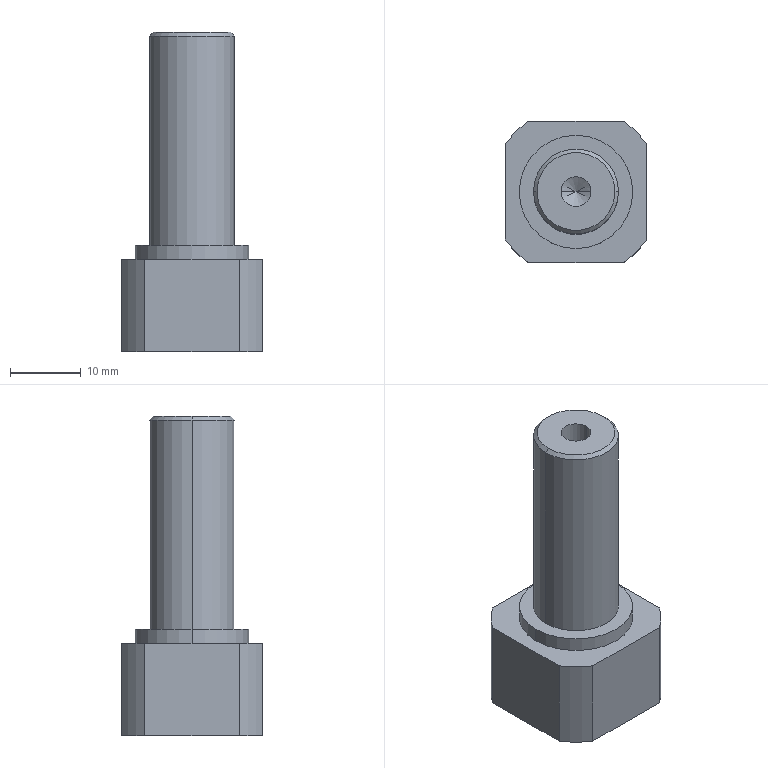Component | SolidWorks | 8TC-A15004-D0-15A-1 | 1 solid | 26 faces | box 20 x 20 x 45 mm | volume 8242 mm3 | cylinder 12 | plane 8 | cone 6 | commonest cylinder face diameters 24 x4 4.2 x2 5 x2 16 x2 12 x2 | material #45
build123d program:
from build123d import *

# Parameters (mm, degrees)
SKETCH2_OUTSIDE_W     = 37.782
SKETCH2_OUTSIDE_H     = 37.782
SKETCH2_OUTSIDE_W_2   = 20
SKETCH2_OUTSIDE_H_2   = 20
CUT_EXTRUDE1_DEPTH    = 40.032
M6_TAPPED_HOLE1_D     = 5
M6_TAPPED_HOLE1_DEPTH = 17
M6_TAPPED_HOLE1_TIP   = 1.502
CHAMFER1_SIZE         = 0.5
SKETCH5_R             = 14.951
CUT_EXTRUDE2_DEPTH    = 3.15
M5_TAPPED_HOLE1_D     = 4.2
M5_TAPPED_HOLE1_DEPTH = 10.4
M5_TAPPED_HOLE1_TIP   = 1.262
CHAMFER2_SIZE         = 0.5


with BuildPart() as part:
    # Sketch1 → Revolve1 (revolve)
    with BuildSketch(Plane.XY, mode=Mode.PRIVATE) as revolve1_sk:
        Polygon((-48.15, 0), (-48.15, 6), (-46.15, 6), (-46.15, 5.7), (-45, 5.7), (-45, 6), (-15, 6), (-15, 8), (-13, 8), (-13, 12), (0, 12), (0, 0), align=None)
    revolve(revolve1_sk.sketch.rotate(Axis((0, 0, 0), (-1, 0, 0)), 90), axis=Axis((0, 0, 0), (-1, 0, 0)))

    # Sketch2 outside → Cut-Extrude1 (cut, through all)
    with BuildSketch(Plane.ZY.offset(13)):
        Rectangle(SKETCH2_OUTSIDE_W, SKETCH2_OUTSIDE_H)
        Rectangle(SKETCH2_OUTSIDE_W_2, SKETCH2_OUTSIDE_H_2, mode=Mode.SUBTRACT)
    extrude(amount=-CUT_EXTRUDE1_DEPTH, mode=Mode.SUBTRACT)

    # M6 Tapped Hole1
    with Locations(Plane(origin=(0, 0, 0), x_dir=(0, 0, -1), z_dir=(1, 0, 0))):
        with Locations((0, 0)):
            Hole(M6_TAPPED_HOLE1_D / 2, depth=M6_TAPPED_HOLE1_DEPTH)
            with Locations((0, 0, -(M6_TAPPED_HOLE1_DEPTH + M6_TAPPED_HOLE1_TIP / 2))):  # 118° drill point
                Cone(0, M6_TAPPED_HOLE1_D / 2, M6_TAPPED_HOLE1_TIP, mode=Mode.SUBTRACT)

    # Chamfer1
    chamfer1_edges = [part.edges().sort_by_distance(p)[0] for p in [
        (-48.15, 0, 6),
    ]]
    chamfer(chamfer1_edges, length=CHAMFER1_SIZE)

    # Sketch5 → Cut-Extrude2 (cut)
    with BuildSketch(Plane.ZY.offset(48.15)):
        Circle(SKETCH5_R)
    extrude(amount=-CUT_EXTRUDE2_DEPTH, mode=Mode.SUBTRACT)

    # M5 Tapped Hole1
    with Locations(Plane.ZY.offset(45)):
        with Locations((0, 0)):
            Hole(M5_TAPPED_HOLE1_D / 2, depth=M5_TAPPED_HOLE1_DEPTH)
            with Locations((0, 0, -(M5_TAPPED_HOLE1_DEPTH + M5_TAPPED_HOLE1_TIP / 2))):  # 118° drill point
                Cone(0, M5_TAPPED_HOLE1_D / 2, M5_TAPPED_HOLE1_TIP, mode=Mode.SUBTRACT)

    # Chamfer2
    chamfer2_edges = [part.edges().sort_by_distance(p)[0] for p in [
        (-45, 0, 6),
    ]]
    chamfer(chamfer2_edges, length=CHAMFER2_SIZE)


solid = part.part

# Placed as in the assembly
solid = solid.moved(Location((29.5, 189.5, 116), (0, 90, 0)))
STEP:
#1=COLOUR_RGB('',0.7922,0.8196,0.9333);
#2=FILL_AREA_STYLE_COLOUR('',#1);
#3=FILL_AREA_STYLE('',(#2));
#4=SURFACE_STYLE_FILL_AREA(#3);
#5=SURFACE_SIDE_STYLE('',(#4));
#6=SURFACE_STYLE_USAGE(.BOTH.,#5);
#7=PRESENTATION_STYLE_ASSIGNMENT((#6));
#8=CARTESIAN_POINT('',(1.378,7.461,6.339));
#9=VERTEX_POINT('',#8);
#10=CARTESIAN_POINT('',(0.9449,7.461,6.339));
#11=VERTEX_POINT('',#10);
#12=CARTESIAN_POINT('',(1.161,7.461,6.339));
#13=DIRECTION('',(0.,0.,1.));
#14=DIRECTION('',(1.,0.,0.));
#15=AXIS2_PLACEMENT_3D('',#12,#13,#14);
#16=CIRCLE('',#15,0.2165);
#17=EDGE_CURVE('',#9,#11,#16,.T.);
#18=ORIENTED_EDGE('',*,*,#17,.F.);
#19=CARTESIAN_POINT('',(1.398,7.461,6.319));
#20=VERTEX_POINT('',#19);
#21=CARTESIAN_POINT('',(1.398,7.461,6.319));
#22=DIRECTION('',(0.7071,0.,-0.7071));
#23=VECTOR('',#22,39.37);
#24=LINE('',#21,#23);
#25=EDGE_CURVE('',#9,#20,#24,.T.);
#26=ORIENTED_EDGE('',*,*,#25,.T.);
#27=CARTESIAN_POINT('',(0.9252,7.461,6.319));
#28=VERTEX_POINT('',#27);
#29=CARTESIAN_POINT('',(1.161,7.461,6.319));
#30=DIRECTION('',(0.,0.,-1.));
#31=DIRECTION('',(1.,0.,0.));
#32=AXIS2_PLACEMENT_3D('',#29,#30,#31);
#33=CIRCLE('',#32,0.2362);
#34=EDGE_CURVE('',#28,#20,#33,.T.);
#35=ORIENTED_EDGE('',*,*,#34,.F.);
#36=CARTESIAN_POINT('',(0.9252,7.461,6.319));
#37=DIRECTION('',(-0.7071,0.,-0.7071));
#38=VECTOR('',#37,39.37);
#39=LINE('',#36,#38);
#40=EDGE_CURVE('',#11,#28,#39,.T.);
#41=ORIENTED_EDGE('',*,*,#40,.F.);
#42=EDGE_LOOP('',(#18,#26,#35,#41));
#43=FACE_OUTER_BOUND('',#42,.T.);
#44=CARTESIAN_POINT('',(1.161,7.461,6.319));
#45=DIRECTION('',(0.,0.,-1.));
#46=DIRECTION('',(-1.,0.,0.));
#47=AXIS2_PLACEMENT_3D('',#44,#45,#46);
#48=CONICAL_SURFACE('',#47,0.2362,0.7854);
#49=ADVANCED_FACE('',(#43),#48,.T.);
#50=CARTESIAN_POINT('',(1.079,7.461,5.929));
#51=VERTEX_POINT('',#50);
#52=CARTESIAN_POINT('',(1.244,7.461,5.929));
#53=VERTEX_POINT('',#52);
#54=CARTESIAN_POINT('',(1.161,7.461,5.929));
#55=DIRECTION('',(0.,0.,1.));
#56=DIRECTION('',(1.,0.,0.));
#57=AXIS2_PLACEMENT_3D('',#54,#55,#56);
#58=CIRCLE('',#57,0.08268);
#59=EDGE_CURVE('',#51,#53,#58,.T.);
#60=ORIENTED_EDGE('',*,*,#59,.F.);
#61=CARTESIAN_POINT('',(1.079,7.461,6.339));
#62=VERTEX_POINT('',#61);
#63=CARTESIAN_POINT('',(1.079,7.461,6.339));
#64=DIRECTION('',(0.,0.,1.));
#65=VECTOR('',#64,39.37);
#66=LINE('',#63,#65);
#67=EDGE_CURVE('',#51,#62,#66,.T.);
#68=ORIENTED_EDGE('',*,*,#67,.T.);
#69=CARTESIAN_POINT('',(1.244,7.461,6.339));
#70=VERTEX_POINT('',#69);
#71=CARTESIAN_POINT('',(1.161,7.461,6.339));
#72=DIRECTION('',(0.,0.,1.));
#73=DIRECTION('',(1.,0.,0.));
#74=AXIS2_PLACEMENT_3D('',#71,#72,#73);
#75=CIRCLE('',#74,0.08268);
#76=EDGE_CURVE('',#62,#70,#75,.T.);
#77=ORIENTED_EDGE('',*,*,#76,.T.);
#78=CARTESIAN_POINT('',(1.244,7.461,6.339));
#79=DIRECTION('',(0.,0.,1.));
#80=VECTOR('',#79,39.37);
#81=LINE('',#78,#80);
#82=EDGE_CURVE('',#53,#70,#81,.T.);
#83=ORIENTED_EDGE('',*,*,#82,.F.);
#84=EDGE_LOOP('',(#60,#68,#77,#83));
#85=FACE_OUTER_BOUND('',#84,.T.);
#86=CARTESIAN_POINT('',(1.161,7.461,6.339));
#87=DIRECTION('',(0.,0.,1.));
#88=DIRECTION('',(1.,0.,0.));
#89=AXIS2_PLACEMENT_3D('',#86,#87,#88);
#90=CYLINDRICAL_SURFACE('',#89,0.08268);
#91=ADVANCED_FACE('',(#85),#90,.F.);
#92=CARTESIAN_POINT('',(1.161,7.461,5.879));
#93=VERTEX_POINT('',#92);
#94=CARTESIAN_POINT('',(1.244,7.461,5.929));
#95=DIRECTION('',(0.8572,0.,0.515));
#96=VECTOR('',#95,39.37);
#97=LINE('',#94,#96);
#98=EDGE_CURVE('',#93,#53,#97,.T.);
#99=ORIENTED_EDGE('',*,*,#98,.F.);
#100=CARTESIAN_POINT('',(1.079,7.461,5.929));
#101=DIRECTION('',(-0.8572,0.,0.515));
#102=VECTOR('',#101,39.37);
#103=LINE('',#100,#102);
#104=EDGE_CURVE('',#93,#51,#103,.T.);
#105=ORIENTED_EDGE('',*,*,#104,.T.);
#106=ORIENTED_EDGE('',*,*,#59,.T.);
#107=EDGE_LOOP('',(#99,#105,#106));
#108=FACE_OUTER_BOUND('',#107,.T.);
#109=CARTESIAN_POINT('',(1.161,7.461,5.929));
#110=DIRECTION('',(0.,0.,1.));
#111=DIRECTION('',(1.,0.,0.));
#112=AXIS2_PLACEMENT_3D('',#109,#110,#111);
#113=CONICAL_SURFACE('',#112,0.08268,1.03);
#114=ADVANCED_FACE('',(#108),#113,.F.);
#115=CARTESIAN_POINT('',(1.26,7.461,5.236));
#116=VERTEX_POINT('',#115);
#117=CARTESIAN_POINT('',(1.063,7.461,5.236));
#118=VERTEX_POINT('',#117);
#119=CARTESIAN_POINT('',(1.161,7.461,5.236));
#120=DIRECTION('',(0.,0.,-1.));
#121=DIRECTION('',(-1.,0.,0.));
#122=AXIS2_PLACEMENT_3D('',#119,#120,#121);
#123=CIRCLE('',#122,0.09843);
#124=EDGE_CURVE('',#116,#118,#123,.T.);
#125=ORIENTED_EDGE('',*,*,#124,.F.);
#126=CARTESIAN_POINT('',(1.26,7.461,4.567));
#127=VERTEX_POINT('',#126);
#128=CARTESIAN_POINT('',(1.26,7.461,4.567));
#129=DIRECTION('',(0.,0.,-1.));
#130=VECTOR('',#129,39.37);
#131=LINE('',#128,#130);
#132=EDGE_CURVE('',#116,#127,#131,.T.);
#133=ORIENTED_EDGE('',*,*,#132,.T.);
#134=CARTESIAN_POINT('',(1.063,7.461,4.567));
#135=VERTEX_POINT('',#134);
#136=CARTESIAN_POINT('',(1.161,7.461,4.567));
#137=DIRECTION('',(0.,0.,-1.));
#138=DIRECTION('',(-1.,0.,0.));
#139=AXIS2_PLACEMENT_3D('',#136,#137,#138);
#140=CIRCLE('',#139,0.09843);
#141=EDGE_CURVE('',#127,#135,#140,.T.);
#142=ORIENTED_EDGE('',*,*,#141,.T.);
#143=CARTESIAN_POINT('',(1.063,7.461,4.567));
#144=DIRECTION('',(0.,0.,-1.));
#145=VECTOR('',#144,39.37);
#146=LINE('',#143,#145);
#147=EDGE_CURVE('',#118,#135,#146,.T.);
#148=ORIENTED_EDGE('',*,*,#147,.F.);
#149=EDGE_LOOP('',(#125,#133,#142,#148));
#150=FACE_OUTER_BOUND('',#149,.T.);
#151=CARTESIAN_POINT('',(1.161,7.461,4.567));
#152=DIRECTION('',(0.,0.,-1.));
#153=DIRECTION('',(-1.,0.,0.));
#154=AXIS2_PLACEMENT_3D('',#151,#152,#153);
#155=CYLINDRICAL_SURFACE('',#154,0.09843);
#156=ADVANCED_FACE('',(#150),#155,.F.);
#157=CARTESIAN_POINT('',(1.161,7.461,5.295));
#158=VERTEX_POINT('',#157);
#159=CARTESIAN_POINT('',(1.063,7.461,5.236));
#160=DIRECTION('',(-0.8572,0.,-0.515));
#161=VECTOR('',#160,39.37);
#162=LINE('',#159,#161);
#163=EDGE_CURVE('',#158,#118,#162,.T.);
#164=ORIENTED_EDGE('',*,*,#163,.F.);
#165=CARTESIAN_POINT('',(1.26,7.461,5.236));
#166=DIRECTION('',(0.8572,0.,-0.515));
#167=VECTOR('',#166,39.37);
#168=LINE('',#165,#167);
#169=EDGE_CURVE('',#158,#116,#168,.T.);
#170=ORIENTED_EDGE('',*,*,#169,.T.);
#171=ORIENTED_EDGE('',*,*,#124,.T.);
#172=EDGE_LOOP('',(#164,#170,#171));
#173=FACE_OUTER_BOUND('',#172,.T.);
#174=CARTESIAN_POINT('',(1.161,7.461,5.236));
#175=DIRECTION('',(0.,0.,-1.));
#176=DIRECTION('',(-1.,0.,0.));
#177=AXIS2_PLACEMENT_3D('',#174,#175,#176);
#178=CONICAL_SURFACE('',#177,0.09843,1.03);
#179=ADVANCED_FACE('',(#173),#178,.F.);
#180=CARTESIAN_POINT('',(0.8465,7.461,5.157));
#181=VERTEX_POINT('',#180);
#182=CARTESIAN_POINT('',(1.476,7.461,5.157));
#183=VERTEX_POINT('',#182);
#184=CARTESIAN_POINT('',(1.161,7.461,5.157));
#185=DIRECTION('',(0.,0.,-1.));
#186=DIRECTION('',(-1.,0.,0.));
#187=AXIS2_PLACEMENT_3D('',#184,#185,#186);
#188=CIRCLE('',#187,0.315);
#189=EDGE_CURVE('',#181,#183,#188,.T.);
#190=ORIENTED_EDGE('',*,*,#189,.T.);
#191=CARTESIAN_POINT('',(1.476,7.461,5.079));
#192=VERTEX_POINT('',#191);
#193=CARTESIAN_POINT('',(1.476,7.461,4.567));
#194=DIRECTION('',(0.,0.,-1.));
#195=VECTOR('',#194,39.37);
#196=LINE('',#193,#195);
#197=EDGE_CURVE('',#183,#192,#196,.T.);
#198=ORIENTED_EDGE('',*,*,#197,.T.);
#199=CARTESIAN_POINT('',(0.8465,7.461,5.079));
#200=VERTEX_POINT('',#199);
#201=CARTESIAN_POINT('',(1.161,7.461,5.079));
#202=DIRECTION('',(0.,0.,-1.));
#203=DIRECTION('',(-1.,0.,0.));
#204=AXIS2_PLACEMENT_3D('',#201,#202,#203);
#205=CIRCLE('',#204,0.315);
#206=EDGE_CURVE('',#200,#192,#205,.T.);
#207=ORIENTED_EDGE('',*,*,#206,.F.);
#208=CARTESIAN_POINT('',(0.8465,7.461,4.567));
#209=DIRECTION('',(0.,0.,-1.));
#210=VECTOR('',#209,39.37);
#211=LINE('',#208,#210);
#212=EDGE_CURVE('',#181,#200,#211,.T.);
#213=ORIENTED_EDGE('',*,*,#212,.F.);
#214=EDGE_LOOP('',(#190,#198,#207,#213));
#215=FACE_OUTER_BOUND('',#214,.T.);
#216=CARTESIAN_POINT('',(1.161,7.461,4.567));
#217=DIRECTION('',(0.,0.,-1.));
#218=DIRECTION('',(-1.,0.,0.));
#219=AXIS2_PLACEMENT_3D('',#216,#217,#218);
#220=CYLINDRICAL_SURFACE('',#219,0.315);
#221=ADVANCED_FACE('',(#215),#220,.T.);
#222=ORIENTED_EDGE('',*,*,#34,.T.);
#223=CARTESIAN_POINT('',(1.398,7.461,5.157));
#224=VERTEX_POINT('',#223);
#225=CARTESIAN_POINT('',(1.398,7.461,4.567));
#226=DIRECTION('',(0.,0.,-1.));
#227=VECTOR('',#226,39.37);
#228=LINE('',#225,#227);
#229=EDGE_CURVE('',#20,#224,#228,.T.);
#230=ORIENTED_EDGE('',*,*,#229,.T.);
#231=CARTESIAN_POINT('',(0.9252,7.461,5.157));
#232=VERTEX_POINT('',#231);
#233=CARTESIAN_POINT('',(1.161,7.461,5.157));
#234=DIRECTION('',(0.,0.,-1.));
#235=DIRECTION('',(-1.,0.,0.));
#236=AXIS2_PLACEMENT_3D('',#233,#234,#235);
#237=CIRCLE('',#236,0.2362);
#238=EDGE_CURVE('',#232,#224,#237,.T.);
#239=ORIENTED_EDGE('',*,*,#238,.F.);
#240=CARTESIAN_POINT('',(0.9252,7.461,4.567));
#241=DIRECTION('',(0.,0.,-1.));
#242=VECTOR('',#241,39.37);
#243=LINE('',#240,#242);
#244=EDGE_CURVE('',#28,#232,#243,.T.);
#245=ORIENTED_EDGE('',*,*,#244,.F.);
#246=EDGE_LOOP('',(#222,#230,#239,#245));
#247=FACE_OUTER_BOUND('',#246,.T.);
#248=CARTESIAN_POINT('',(1.161,7.461,4.567));
#249=DIRECTION('',(0.,0.,-1.));
#250=DIRECTION('',(-1.,0.,0.));
#251=AXIS2_PLACEMENT_3D('',#248,#249,#250);
#252=CYLINDRICAL_SURFACE('',#251,0.2362);
#253=ADVANCED_FACE('',(#247),#252,.T.);
#254=ORIENTED_EDGE('',*,*,#206,.T.);
#255=CARTESIAN_POINT('',(1.161,7.461,5.079));
#256=DIRECTION('',(0.,0.,-1.));
#257=DIRECTION('',(-1.,0.,0.));
#258=AXIS2_PLACEMENT_3D('',#255,#256,#257);
#259=CIRCLE('',#258,0.315);
#260=EDGE_CURVE('',#192,#200,#259,.T.);
#261=ORIENTED_EDGE('',*,*,#260,.T.);
#262=EDGE_LOOP('',(#254,#261));
#263=FACE_BOUND('',#262,.T.);
#264=CARTESIAN_POINT('',(1.555,7.199,5.079));
#265=VERTEX_POINT('',#264);
#266=CARTESIAN_POINT('',(1.423,7.067,5.079));
#267=VERTEX_POINT('',#266);
#268=CARTESIAN_POINT('',(1.161,7.461,5.079));
#269=DIRECTION('',(0.,0.,-1.));
#270=DIRECTION('',(-1.,0.,0.));
#271=AXIS2_PLACEMENT_3D('',#268,#269,#270);
#272=CIRCLE('',#271,0.4724);
#273=EDGE_CURVE('',#265,#267,#272,.T.);
#274=ORIENTED_EDGE('',*,*,#273,.F.);
#275=CARTESIAN_POINT('',(1.555,7.722,5.079));
#276=VERTEX_POINT('',#275);
#277=CARTESIAN_POINT('',(1.555,7.067,5.079));
#278=DIRECTION('',(0.,1.,0.));
#279=VECTOR('',#278,39.37);
#280=LINE('',#277,#279);
#281=EDGE_CURVE('',#265,#276,#280,.T.);
#282=ORIENTED_EDGE('',*,*,#281,.T.);
#283=CARTESIAN_POINT('',(1.423,7.854,5.079));
#284=VERTEX_POINT('',#283);
#285=CARTESIAN_POINT('',(1.161,7.461,5.079));
#286=DIRECTION('',(0.,0.,-1.));
#287=DIRECTION('',(-1.,0.,0.));
#288=AXIS2_PLACEMENT_3D('',#285,#286,#287);
#289=CIRCLE('',#288,0.4724);
#290=EDGE_CURVE('',#284,#276,#289,.T.);
#291=ORIENTED_EDGE('',*,*,#290,.F.);
#292=CARTESIAN_POINT('',(0.9003,7.854,5.079));
#293=VERTEX_POINT('',#292);
#294=CARTESIAN_POINT('',(0.7677,7.854,5.079));
#295=DIRECTION('',(-1.,0.,0.));
#296=VECTOR('',#295,39.37);
#297=LINE('',#294,#296);
#298=EDGE_CURVE('',#284,#293,#297,.T.);
#299=ORIENTED_EDGE('',*,*,#298,.T.);
#300=CARTESIAN_POINT('',(0.7677,7.722,5.079));
#301=VERTEX_POINT('',#300);
#302=CARTESIAN_POINT('',(1.161,7.461,5.079));
#303=DIRECTION('',(0.,0.,-1.));
#304=DIRECTION('',(-1.,0.,0.));
#305=AXIS2_PLACEMENT_3D('',#302,#303,#304);
#306=CIRCLE('',#305,0.4724);
#307=EDGE_CURVE('',#301,#293,#306,.T.);
#308=ORIENTED_EDGE('',*,*,#307,.F.);
#309=CARTESIAN_POINT('',(0.7677,7.199,5.079));
#310=VERTEX_POINT('',#309);
#311=CARTESIAN_POINT('',(0.7677,7.067,5.079));
#312=DIRECTION('',(0.,-1.,0.));
#313=VECTOR('',#312,39.37);
#314=LINE('',#311,#313);
#315=EDGE_CURVE('',#301,#310,#314,.T.);
#316=ORIENTED_EDGE('',*,*,#315,.T.);
#317=CARTESIAN_POINT('',(0.9003,7.067,5.079));
#318=VERTEX_POINT('',#317);
#319=CARTESIAN_POINT('',(1.161,7.461,5.079));
#320=DIRECTION('',(0.,0.,-1.));
#321=DIRECTION('',(-1.,0.,0.));
#322=AXIS2_PLACEMENT_3D('',#319,#320,#321);
#323=CIRCLE('',#322,0.4724);
#324=EDGE_CURVE('',#318,#310,#323,.T.);
#325=ORIENTED_EDGE('',*,*,#324,.F.);
#326=CARTESIAN_POINT('',(0.7677,7.067,5.079));
#327=DIRECTION('',(1.,0.,0.));
#328=VECTOR('',#327,39.37);
#329=LINE('',#326,#328);
#330=EDGE_CURVE('',#318,#267,#329,.T.);
#331=ORIENTED_EDGE('',*,*,#330,.T.);
#332=EDGE_LOOP('',(#274,#282,#291,#299,#308,#316,#325,#331));
#333=FACE_OUTER_BOUND('',#332,.T.);
#334=CARTESIAN_POINT('',(1.161,7.776,5.079));
#335=DIRECTION('',(0.,0.,1.));
#336=DIRECTION('',(1.,0.,0.));
#337=AXIS2_PLACEMENT_3D('',#334,#335,#336);
#338=PLANE('',#337);
#339=ADVANCED_FACE('',(#263,#333),#338,.T.);
#340=CARTESIAN_POINT('',(1.555,7.199,4.567));
#341=VERTEX_POINT('',#340);
#342=CARTESIAN_POINT('',(1.423,7.067,4.567));
#343=VERTEX_POINT('',#342);
#344=CARTESIAN_POINT('',(1.161,7.461,4.567));
#345=DIRECTION('',(0.,0.,-1.));
#346=DIRECTION('',(-1.,0.,0.));
#347=AXIS2_PLACEMENT_3D('',#344,#345,#346);
#348=CIRCLE('',#347,0.4724);
#349=EDGE_CURVE('',#341,#343,#348,.T.);
#350=ORIENTED_EDGE('',*,*,#349,.F.);
#351=CARTESIAN_POINT('',(1.555,7.199,4.567));
#352=DIRECTION('',(0.,0.,1.));
#353=VECTOR('',#352,39.37);
#354=LINE('',#351,#353);
#355=EDGE_CURVE('',#341,#265,#354,.T.);
#356=ORIENTED_EDGE('',*,*,#355,.T.);
#357=ORIENTED_EDGE('',*,*,#273,.T.);
#358=CARTESIAN_POINT('',(1.423,7.067,4.567));
#359=DIRECTION('',(0.,0.,-1.));
#360=VECTOR('',#359,39.37);
#361=LINE('',#358,#360);
#362=EDGE_CURVE('',#267,#343,#361,.T.);
#363=ORIENTED_EDGE('',*,*,#362,.T.);
#364=EDGE_LOOP('',(#350,#356,#357,#363));
#365=FACE_OUTER_BOUND('',#364,.T.);
#366=CARTESIAN_POINT('',(1.161,7.461,4.567));
#367=DIRECTION('',(0.,0.,-1.));
#368=DIRECTION('',(-1.,0.,0.));
#369=AXIS2_PLACEMENT_3D('',#366,#367,#368);
#370=CYLINDRICAL_SURFACE('',#369,0.4724);
#371=ADVANCED_FACE('',(#365),#370,.T.);
#372=ORIENTED_EDGE('',*,*,#290,.T.);
#373=CARTESIAN_POINT('',(1.555,7.722,4.567));
#374=VERTEX_POINT('',#373);
#375=CARTESIAN_POINT('',(1.555,7.722,4.567));
#376=DIRECTION('',(0.,0.,-1.));
#377=VECTOR('',#376,39.37);
#378=LINE('',#375,#377);
#379=EDGE_CURVE('',#276,#374,#378,.T.);
#380=ORIENTED_EDGE('',*,*,#379,.T.);
#381=CARTESIAN_POINT('',(1.423,7.854,4.567));
#382=VERTEX_POINT('',#381);
#383=CARTESIAN_POINT('',(1.161,7.461,4.567));
#384=DIRECTION('',(0.,0.,-1.));
#385=DIRECTION('',(-1.,0.,0.));
#386=AXIS2_PLACEMENT_3D('',#383,#384,#385);
#387=CIRCLE('',#386,0.4724);
#388=EDGE_CURVE('',#382,#374,#387,.T.);
#389=ORIENTED_EDGE('',*,*,#388,.F.);
#390=CARTESIAN_POINT('',(1.423,7.854,4.567));
#391=DIRECTION('',(0.,0.,1.));
#392=VECTOR('',#391,39.37);
#393=LINE('',#390,#392);
#394=EDGE_CURVE('',#382,#284,#393,.T.);
#395=ORIENTED_EDGE('',*,*,#394,.T.);
#396=EDGE_LOOP('',(#372,#380,#389,#395));
#397=FACE_OUTER_BOUND('',#396,.T.);
#398=CARTESIAN_POINT('',(1.161,7.461,4.567));
#399=DIRECTION('',(0.,0.,-1.));
#400=DIRECTION('',(-1.,0.,0.));
#401=AXIS2_PLACEMENT_3D('',#398,#399,#400);
#402=CYLINDRICAL_SURFACE('',#401,0.4724);
#403=ADVANCED_FACE('',(#397),#402,.T.);
#404=CARTESIAN_POINT('',(0.9003,7.067,4.567));
#405=VERTEX_POINT('',#404);
#406=CARTESIAN_POINT('',(0.7677,7.199,4.567));
#407=VERTEX_POINT('',#406);
#408=CARTESIAN_POINT('',(1.161,7.461,4.567));
#409=DIRECTION('',(0.,0.,-1.));
#410=DIRECTION('',(-1.,0.,0.));
#411=AXIS2_PLACEMENT_3D('',#408,#409,#410);
#412=CIRCLE('',#411,0.4724);
#413=EDGE_CURVE('',#405,#407,#412,.T.);
#414=ORIENTED_EDGE('',*,*,#413,.F.);
#415=CARTESIAN_POINT('',(0.9003,7.067,4.567));
#416=DIRECTION('',(0.,0.,1.));
#417=VECTOR('',#416,39.37);
#418=LINE('',#415,#417);
#419=EDGE_CURVE('',#405,#318,#418,.T.);
#420=ORIENTED_EDGE('',*,*,#419,.T.);
#421=ORIENTED_EDGE('',*,*,#324,.T.);
#422=CARTESIAN_POINT('',(0.7677,7.199,4.567));
#423=DIRECTION('',(0.,0.,-1.));
#424=VECTOR('',#423,39.37);
#425=LINE('',#422,#424);
#426=EDGE_CURVE('',#310,#407,#425,.T.);
#427=ORIENTED_EDGE('',*,*,#426,.T.);
#428=EDGE_LOOP('',(#414,#420,#421,#427));
#429=FACE_OUTER_BOUND('',#428,.T.);
#430=CARTESIAN_POINT('',(1.161,7.461,4.567));
#431=DIRECTION('',(0.,0.,-1.));
#432=DIRECTION('',(-1.,0.,0.));
#433=AXIS2_PLACEMENT_3D('',#430,#431,#432);
#434=CYLINDRICAL_SURFACE('',#433,0.4724);
#435=ADVANCED_FACE('',(#429),#434,.T.);
#436=CARTESIAN_POINT('',(0.7677,7.722,4.567));
#437=VERTEX_POINT('',#436);
#438=CARTESIAN_POINT('',(0.9003,7.854,4.567));
#439=VERTEX_POINT('',#438);
#440=CARTESIAN_POINT('',(1.161,7.461,4.567));
#441=DIRECTION('',(0.,0.,-1.));
#442=DIRECTION('',(-1.,0.,0.));
#443=AXIS2_PLACEMENT_3D('',#440,#441,#442);
#444=CIRCLE('',#443,0.4724);
#445=EDGE_CURVE('',#437,#439,#444,.T.);
#446=ORIENTED_EDGE('',*,*,#445,.F.);
#447=CARTESIAN_POINT('',(0.7677,7.722,4.567));
#448=DIRECTION('',(0.,0.,1.));
#449=VECTOR('',#448,39.37);
#450=LINE('',#447,#449);
#451=EDGE_CURVE('',#437,#301,#450,.T.);
#452=ORIENTED_EDGE('',*,*,#451,.T.);
#453=ORIENTED_EDGE('',*,*,#307,.T.);
#454=CARTESIAN_POINT('',(0.9003,7.854,4.567));
#455=DIRECTION('',(0.,0.,-1.));
#456=VECTOR('',#455,39.37);
#457=LINE('',#454,#456);
#458=EDGE_CURVE('',#293,#439,#457,.T.);
#459=ORIENTED_EDGE('',*,*,#458,.T.);
#460=EDGE_LOOP('',(#446,#452,#453,#459));
#461=FACE_OUTER_BOUND('',#460,.T.);
#462=CARTESIAN_POINT('',(1.161,7.461,4.567));
#463=DIRECTION('',(0.,0.,-1.));
#464=DIRECTION('',(-1.,0.,0.));
#465=AXIS2_PLACEMENT_3D('',#462,#463,#464);
#466=CYLINDRICAL_SURFACE('',#465,0.4724);
#467=ADVANCED_FACE('',(#461),#466,.T.);
#468=CARTESIAN_POINT('',(1.161,7.461,4.567));
#469=DIRECTION('',(0.,0.,-1.));
#470=DIRECTION('',(-1.,0.,0.));
#471=AXIS2_PLACEMENT_3D('',#468,#469,#470);
#472=CIRCLE('',#471,0.09843);
#473=EDGE_CURVE('',#135,#127,#472,.T.);
#474=ORIENTED_EDGE('',*,*,#473,.F.);
#475=ORIENTED_EDGE('',*,*,#141,.F.);
#476=EDGE_LOOP('',(#474,#475));
#477=FACE_BOUND('',#476,.T.);
#478=ORIENTED_EDGE('',*,*,#388,.T.);
#479=CARTESIAN_POINT('',(1.555,7.933,4.567));
#480=DIRECTION('',(0.,-1.,0.));
#481=VECTOR('',#480,39.37);
#482=LINE('',#479,#481);
#483=EDGE_CURVE('',#374,#341,#482,.T.);
#484=ORIENTED_EDGE('',*,*,#483,.T.);
#485=ORIENTED_EDGE('',*,*,#349,.T.);
#486=CARTESIAN_POINT('',(1.161,7.067,4.567));
#487=DIRECTION('',(-1.,0.,0.));
#488=VECTOR('',#487,39.37);
#489=LINE('',#486,#488);
#490=EDGE_CURVE('',#343,#405,#489,.T.);
#491=ORIENTED_EDGE('',*,*,#490,.T.);
#492=ORIENTED_EDGE('',*,*,#413,.T.);
#493=CARTESIAN_POINT('',(0.7677,7.933,4.567));
#494=DIRECTION('',(0.,1.,0.));
#495=VECTOR('',#494,39.37);
#496=LINE('',#493,#495);
#497=EDGE_CURVE('',#407,#437,#496,.T.);
#498=ORIENTED_EDGE('',*,*,#497,.T.);
#499=ORIENTED_EDGE('',*,*,#445,.T.);
#500=CARTESIAN_POINT('',(1.161,7.854,4.567));
#501=DIRECTION('',(1.,0.,0.));
#502=VECTOR('',#501,39.37);
#503=LINE('',#500,#502);
#504=EDGE_CURVE('',#439,#382,#503,.T.);
#505=ORIENTED_EDGE('',*,*,#504,.T.);
#506=EDGE_LOOP('',(#478,#484,#485,#491,#492,#498,#499,#505));
#507=FACE_OUTER_BOUND('',#506,.T.);
#508=CARTESIAN_POINT('',(1.161,7.933,4.567));
#509=DIRECTION('',(0.,0.,-1.));
#510=DIRECTION('',(-1.,0.,0.));
#511=AXIS2_PLACEMENT_3D('',#508,#509,#510);
#512=PLANE('',#511);
#513=ADVANCED_FACE('',(#477,#507),#512,.T.);
#514=CARTESIAN_POINT('',(1.161,7.461,6.339));
#515=DIRECTION('',(0.,0.,1.));
#516=DIRECTION('',(1.,0.,0.));
#517=AXIS2_PLACEMENT_3D('',#514,#515,#516);
#518=CIRCLE('',#517,0.2165);
#519=EDGE_CURVE('',#11,#9,#518,.T.);
#520=ORIENTED_EDGE('',*,*,#519,.T.);
#521=ORIENTED_EDGE('',*,*,#17,.T.);
#522=EDGE_LOOP('',(#520,#521));
#523=FACE_OUTER_BOUND('',#522,.T.);
#524=CARTESIAN_POINT('',(1.161,7.461,6.339));
#525=DIRECTION('',(0.,0.,1.));
#526=DIRECTION('',(1.,0.,0.));
#527=AXIS2_PLACEMENT_3D('',#524,#525,#526);
#528=CIRCLE('',#527,0.08268);
#529=EDGE_CURVE('',#70,#62,#528,.T.);
#530=ORIENTED_EDGE('',*,*,#529,.F.);
#531=ORIENTED_EDGE('',*,*,#76,.F.);
#532=EDGE_LOOP('',(#530,#531));
#533=FACE_BOUND('',#532,.T.);
#534=CARTESIAN_POINT('',(1.161,7.685,6.339));
#535=DIRECTION('',(0.,0.,1.));
#536=DIRECTION('',(1.,0.,0.));
#537=AXIS2_PLACEMENT_3D('',#534,#535,#536);
#538=PLANE('',#537);
#539=ADVANCED_FACE('',(#523,#533),#538,.T.);
#540=ORIENTED_EDGE('',*,*,#229,.F.);
#541=CARTESIAN_POINT('',(1.161,7.461,6.319));
#542=DIRECTION('',(0.,0.,-1.));
#543=DIRECTION('',(1.,0.,0.));
#544=AXIS2_PLACEMENT_3D('',#541,#542,#543);
#545=CIRCLE('',#544,0.2362);
#546=EDGE_CURVE('',#20,#28,#545,.T.);
#547=ORIENTED_EDGE('',*,*,#546,.T.);
#548=ORIENTED_EDGE('',*,*,#244,.T.);
#549=CARTESIAN_POINT('',(1.161,7.461,5.157));
#550=DIRECTION('',(0.,0.,-1.));
#551=DIRECTION('',(-1.,0.,0.));
#552=AXIS2_PLACEMENT_3D('',#549,#550,#551);
#553=CIRCLE('',#552,0.2362);
#554=EDGE_CURVE('',#224,#232,#553,.T.);
#555=ORIENTED_EDGE('',*,*,#554,.F.);
#556=EDGE_LOOP('',(#540,#547,#548,#555));
#557=FACE_OUTER_BOUND('',#556,.T.);
#558=CARTESIAN_POINT('',(1.161,7.461,4.567));
#559=DIRECTION('',(0.,0.,-1.));
#560=DIRECTION('',(-1.,0.,0.));
#561=AXIS2_PLACEMENT_3D('',#558,#559,#560);
#562=CYLINDRICAL_SURFACE('',#561,0.2362);
#563=ADVANCED_FACE('',(#557),#562,.T.);
#564=ORIENTED_EDGE('',*,*,#238,.T.);
#565=ORIENTED_EDGE('',*,*,#554,.T.);
#566=EDGE_LOOP('',(#564,#565));
#567=FACE_BOUND('',#566,.T.);
#568=ORIENTED_EDGE('',*,*,#189,.F.);
#569=CARTESIAN_POINT('',(1.161,7.461,5.157));
#570=DIRECTION('',(0.,0.,-1.));
#571=DIRECTION('',(-1.,0.,0.));
#572=AXIS2_PLACEMENT_3D('',#569,#570,#571);
#573=CIRCLE('',#572,0.315);
#574=EDGE_CURVE('',#183,#181,#573,.T.);
#575=ORIENTED_EDGE('',*,*,#574,.F.);
#576=EDGE_LOOP('',(#568,#575));
#577=FACE_OUTER_BOUND('',#576,.T.);
#578=CARTESIAN_POINT('',(1.161,7.697,5.157));
#579=DIRECTION('',(0.,0.,1.));
#580=DIRECTION('',(1.,0.,0.));
#581=AXIS2_PLACEMENT_3D('',#578,#579,#580);
#582=PLANE('',#581);
#583=ADVANCED_FACE('',(#567,#577),#582,.T.);
#584=ORIENTED_EDGE('',*,*,#197,.F.);
#585=ORIENTED_EDGE('',*,*,#574,.T.);
#586=ORIENTED_EDGE('',*,*,#212,.T.);
#587=ORIENTED_EDGE('',*,*,#260,.F.);
#588=EDGE_LOOP('',(#584,#585,#586,#587));
#589=FACE_OUTER_BOUND('',#588,.T.);
#590=CARTESIAN_POINT('',(1.161,7.461,4.567));
#591=DIRECTION('',(0.,0.,-1.));
#592=DIRECTION('',(-1.,0.,0.));
#593=AXIS2_PLACEMENT_3D('',#590,#591,#592);
#594=CYLINDRICAL_SURFACE('',#593,0.315);
#595=ADVANCED_FACE('',(#589),#594,.T.);
#596=ORIENTED_EDGE('',*,*,#504,.F.);
#597=ORIENTED_EDGE('',*,*,#458,.F.);
#598=ORIENTED_EDGE('',*,*,#298,.F.);
#599=ORIENTED_EDGE('',*,*,#394,.F.);
#600=EDGE_LOOP('',(#596,#597,#598,#599));
#601=FACE_OUTER_BOUND('',#600,.T.);
#602=CARTESIAN_POINT('',(0.7677,7.854,4.567));
#603=DIRECTION('',(0.,1.,0.));
#604=DIRECTION('',(1.,0.,0.));
#605=AXIS2_PLACEMENT_3D('',#602,#603,#604);
#606=PLANE('',#605);
#607=ADVANCED_FACE('',(#601),#606,.T.);
#608=ORIENTED_EDGE('',*,*,#497,.F.);
#609=ORIENTED_EDGE('',*,*,#426,.F.);
#610=ORIENTED_EDGE('',*,*,#315,.F.);
#611=ORIENTED_EDGE('',*,*,#451,.F.);
#612=EDGE_LOOP('',(#608,#609,#610,#611));
#613=FACE_OUTER_BOUND('',#612,.T.);
#614=CARTESIAN_POINT('',(0.7677,7.067,4.567));
#615=DIRECTION('',(-1.,0.,0.));
#616=DIRECTION('',(0.,0.,1.));
#617=AXIS2_PLACEMENT_3D('',#614,#615,#616);
#618=PLANE('',#617);
#619=ADVANCED_FACE('',(#613),#618,.T.);
#620=ORIENTED_EDGE('',*,*,#490,.F.);
#621=ORIENTED_EDGE('',*,*,#362,.F.);
#622=ORIENTED_EDGE('',*,*,#330,.F.);
#623=ORIENTED_EDGE('',*,*,#419,.F.);
#624=EDGE_LOOP('',(#620,#621,#622,#623));
#625=FACE_OUTER_BOUND('',#624,.T.);
#626=CARTESIAN_POINT('',(0.7677,7.067,4.567));
#627=DIRECTION('',(0.,-1.,0.));
#628=DIRECTION('',(-1.,0.,0.));
#629=AXIS2_PLACEMENT_3D('',#626,#627,#628);
#630=PLANE('',#629);
#631=ADVANCED_FACE('',(#625),#630,.T.);
#632=ORIENTED_EDGE('',*,*,#483,.F.);
#633=ORIENTED_EDGE('',*,*,#379,.F.);
#634=ORIENTED_EDGE('',*,*,#281,.F.);
#635=ORIENTED_EDGE('',*,*,#355,.F.);
#636=EDGE_LOOP('',(#632,#633,#634,#635));
#637=FACE_OUTER_BOUND('',#636,.T.);
#638=CARTESIAN_POINT('',(1.555,7.067,4.567));
#639=DIRECTION('',(1.,0.,0.));
#640=DIRECTION('',(0.,0.,-1.));
#641=AXIS2_PLACEMENT_3D('',#638,#639,#640);
#642=PLANE('',#641);
#643=ADVANCED_FACE('',(#637),#642,.T.);
#644=ORIENTED_EDGE('',*,*,#169,.F.);
#645=ORIENTED_EDGE('',*,*,#163,.T.);
#646=CARTESIAN_POINT('',(1.161,7.461,5.236));
#647=DIRECTION('',(0.,0.,-1.));
#648=DIRECTION('',(-1.,0.,0.));
#649=AXIS2_PLACEMENT_3D('',#646,#647,#648);
#650=CIRCLE('',#649,0.09843);
#651=EDGE_CURVE('',#118,#116,#650,.T.);
#652=ORIENTED_EDGE('',*,*,#651,.T.);
#653=EDGE_LOOP('',(#644,#645,#652));
#654=FACE_OUTER_BOUND('',#653,.T.);
#655=CARTESIAN_POINT('',(1.161,7.461,5.236));
#656=DIRECTION('',(0.,0.,-1.));
#657=DIRECTION('',(-1.,0.,0.));
#658=AXIS2_PLACEMENT_3D('',#655,#656,#657);
#659=CONICAL_SURFACE('',#658,0.09843,1.03);
#660=ADVANCED_FACE('',(#654),#659,.F.);
#661=ORIENTED_EDGE('',*,*,#132,.F.);
#662=ORIENTED_EDGE('',*,*,#651,.F.);
#663=ORIENTED_EDGE('',*,*,#147,.T.);
#664=ORIENTED_EDGE('',*,*,#473,.T.);
#665=EDGE_LOOP('',(#661,#662,#663,#664));
#666=FACE_OUTER_BOUND('',#665,.T.);
#667=CARTESIAN_POINT('',(1.161,7.461,4.567));
#668=DIRECTION('',(0.,0.,-1.));
#669=DIRECTION('',(-1.,0.,0.));
#670=AXIS2_PLACEMENT_3D('',#667,#668,#669);
#671=CYLINDRICAL_SURFACE('',#670,0.09843);
#672=ADVANCED_FACE('',(#666),#671,.F.);
#673=ORIENTED_EDGE('',*,*,#104,.F.);
#674=ORIENTED_EDGE('',*,*,#98,.T.);
#675=CARTESIAN_POINT('',(1.161,7.461,5.929));
#676=DIRECTION('',(0.,0.,1.));
#677=DIRECTION('',(1.,0.,0.));
#678=AXIS2_PLACEMENT_3D('',#675,#676,#677);
#679=CIRCLE('',#678,0.08268);
#680=EDGE_CURVE('',#53,#51,#679,.T.);
#681=ORIENTED_EDGE('',*,*,#680,.T.);
#682=EDGE_LOOP('',(#673,#674,#681));
#683=FACE_OUTER_BOUND('',#682,.T.);
#684=CARTESIAN_POINT('',(1.161,7.461,5.929));
#685=DIRECTION('',(0.,0.,1.));
#686=DIRECTION('',(1.,0.,0.));
#687=AXIS2_PLACEMENT_3D('',#684,#685,#686);
#688=CONICAL_SURFACE('',#687,0.08268,1.03);
#689=ADVANCED_FACE('',(#683),#688,.F.);
#690=ORIENTED_EDGE('',*,*,#67,.F.);
#691=ORIENTED_EDGE('',*,*,#680,.F.);
#692=ORIENTED_EDGE('',*,*,#82,.T.);
#693=ORIENTED_EDGE('',*,*,#529,.T.);
#694=EDGE_LOOP('',(#690,#691,#692,#693));
#695=FACE_OUTER_BOUND('',#694,.T.);
#696=CARTESIAN_POINT('',(1.161,7.461,6.339));
#697=DIRECTION('',(0.,0.,1.));
#698=DIRECTION('',(1.,0.,0.));
#699=AXIS2_PLACEMENT_3D('',#696,#697,#698);
#700=CYLINDRICAL_SURFACE('',#699,0.08268);
#701=ADVANCED_FACE('',(#695),#700,.F.);
#702=ORIENTED_EDGE('',*,*,#25,.F.);
#703=ORIENTED_EDGE('',*,*,#519,.F.);
#704=ORIENTED_EDGE('',*,*,#40,.T.);
#705=ORIENTED_EDGE('',*,*,#546,.F.);
#706=EDGE_LOOP('',(#702,#703,#704,#705));
#707=FACE_OUTER_BOUND('',#706,.T.);
#708=CARTESIAN_POINT('',(1.161,7.461,6.319));
#709=DIRECTION('',(0.,0.,-1.));
#710=DIRECTION('',(-1.,0.,0.));
#711=AXIS2_PLACEMENT_3D('',#708,#709,#710);
#712=CONICAL_SURFACE('',#711,0.2362,0.7854);
#713=ADVANCED_FACE('',(#707),#712,.T.);
#714=CLOSED_SHELL('',(#49,#91,#114,#156,#179,#221,#253,#339,#371,#403,#435,#467,#513,#539,#563,#583,#595,#607,#619,#631,#643,#660,#672,#689,#701,#713));
#715=MANIFOLD_SOLID_BREP('',#714);
#716=STYLED_ITEM('',(#7),#715);
#717=(LENGTH_UNIT()NAMED_UNIT(*)SI_UNIT($,.METRE.));
#718=LENGTH_MEASURE_WITH_UNIT(LENGTH_MEASURE(0.0254),#717);
#719=DIMENSIONAL_EXPONENTS(1.,0.,0.,0.,0.,0.,0.);
#720=(CONVERSION_BASED_UNIT('',#718)LENGTH_UNIT()NAMED_UNIT(#719));
#721=UNCERTAINTY_MEASURE_WITH_UNIT(LENGTH_MEASURE(0.00001),#720,'','');
#722=(NAMED_UNIT(*)PLANE_ANGLE_UNIT()SI_UNIT($,.RADIAN.));
#723=(NAMED_UNIT(*)SI_UNIT($,.STERADIAN.)SOLID_ANGLE_UNIT());
#724=(GEOMETRIC_REPRESENTATION_CONTEXT(3)GLOBAL_UNCERTAINTY_ASSIGNED_CONTEXT((#721))GLOBAL_UNIT_ASSIGNED_CONTEXT((#720,#722,#723))REPRESENTATION_CONTEXT('',''));
#725=MECHANICAL_DESIGN_GEOMETRIC_PRESENTATION_REPRESENTATION('',(#716),#724);
#726=CARTESIAN_POINT('',(0.,0.,0.));
#727=DIRECTION('',(0.,0.,1.));
#728=DIRECTION('',(1.,0.,0.));
#729=AXIS2_PLACEMENT_3D('',#726,#727,#728);
#730=(LENGTH_UNIT()NAMED_UNIT(*)SI_UNIT($,.METRE.));
#731=LENGTH_MEASURE_WITH_UNIT(LENGTH_MEASURE(0.0254),#730);
#732=DIMENSIONAL_EXPONENTS(1.,0.,0.,0.,0.,0.,0.);
#733=(CONVERSION_BASED_UNIT('',#731)LENGTH_UNIT()NAMED_UNIT(#732));
#734=UNCERTAINTY_MEASURE_WITH_UNIT(LENGTH_MEASURE(0.00001),#733,'','');
#735=(NAMED_UNIT(*)PLANE_ANGLE_UNIT()SI_UNIT($,.RADIAN.));
#736=(NAMED_UNIT(*)SI_UNIT($,.STERADIAN.)SOLID_ANGLE_UNIT());
#737=(GEOMETRIC_REPRESENTATION_CONTEXT(3)GLOBAL_UNCERTAINTY_ASSIGNED_CONTEXT((#734))GLOBAL_UNIT_ASSIGNED_CONTEXT((#733,#735,#736))REPRESENTATION_CONTEXT('',''));
#738=ADVANCED_BREP_SHAPE_REPRESENTATION('',(#715,#729),#737);
#739=PRESENTATION_LAYER_ASSIGNMENT('','',(#716));